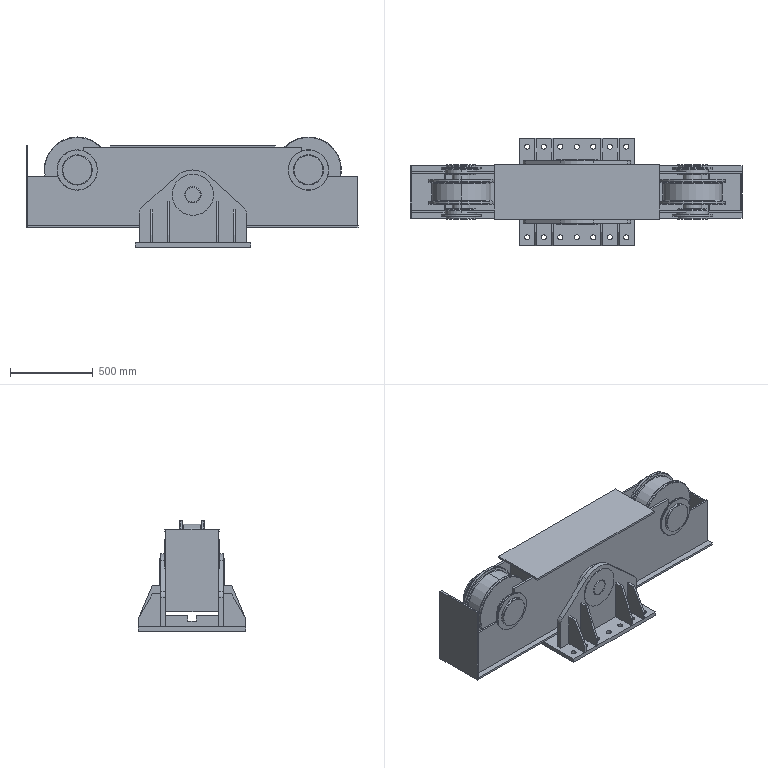Assembly | SolidWorks | mm | 35 component files | 35 solids | 454 faces | box 2010 x 650 x 667 mm | volume 110536923 mm3 | plane 220 | cylinder 134 | torus 72 | cone 28 | commonest cylinder face diameters 100 x30 31 x28 250 x16 195 x14 180 x8 245 x8 240 x8 112 x8
Bill of materials:
700X650X25 | 1 | Plain Carbon Steel | Thin, nearly square flat plate with a single row of seven evenly spaced round through-holes along each of two opposite edges (14 holes total).
Axis | 1 | Plain Carbon Steel | Solid round cylinder (pin or rod shape) with small chamfers or edge breaks at both flat ends.
BottomCover | 1 | Plain Carbon Steel | Thin, plain rectangular flat plate or sheet with no visible holes or cutouts.
Cover1 | 1 | Plain Carbon Steel | Thin, plain rectangular flat plate, taller than it is wide, with no visible features.
Cover2 | 1 | Plain Carbon Steel | Thin, plain rectangular flat plate, close to square, with no visible features. Its thickness ratio is somewhat larger than unnamed part.
FlangeRib1 | 4 | Plain Carbon Steel | Flat plate with a four-sided outline: three square corners and one side cut at an angle, giving a trapezoid with a short vertical edge at the low end.
FlangeRib2 | 4 | Plain Carbon Steel | Flat trapezoidal plate like unnamed part: a straight top, base and one vertical side, plus a long slanted edge that ends in a short vertical edge. It is narrower and slightly steeper than that part.
RibPlate1 | 2 | Plain Carbon Steel | Rectangular flat bar or strip, long compared with its height, with a moderate thickness and no visible holes.
RibPlate2 | 4 | Plain Carbon Steel | Very thin, plain rectangular sheet or plate, taller than it is wide, with no visible features.
SidePlate | 2 | Plain Carbon Steel | Thin, long flat strip with a narrower raised centre section. At each step between the wide and narrow sections there is a rounded, keyhole-like notch, and there is one small round through-hole in the middle.
Support1 | 2 | Plain Carbon Steel | Flat tab or lug plate: a rectangular base with two angled sides rising to a rounded top, small rounded shoulder corners, and one round through-hole near the top.
Support2 | 2 | Plain Carbon Steel | Thin flat ring (washer-like annulus) with a concentric central through-hole.
Support3 | 4 | Plain Carbon Steel | Thin flat circular ring (plain washer-like annulus) with a concentric through-hole; plain flat faces, square edges.
Support4 | 2 | Plain Carbon Steel | Flat circular ring with a concentric through-hole, like part-9d640c60 but visibly thicker; plain flat faces.
Support5 | 1 | Plain Carbon Steel | Rectangular prismatic bar with one rectangular notch cut across its full width at mid-length on one long face.
TopCover | 1 | Plain Carbon Steel | Thin flat rectangular strip or plate with plain rectangular outline; no holes or cutouts visible.
WheelFrom | 2 | Plain Carbon Steel | Rotationally symmetric spool or flanged-roller shape: a central cylindrical drum between two thin end flanges, with a smaller stepped hub sticking out on each side. Each hub ends in a flanged collar.
Mates:
1. coincident | TopCover-1 face at (1250.579, 1256.349, 1665.088) dir (0, 0, 1) | SidePlate-1 face at (2250.579, 1381.349, 1665.088) dir (0, 0, -1)
2. distance | SidePlate-1 face at (1950.579, 1381.349, 2003.088) dir (0, 1, 0) | TopCover-1 face at (250.579, 1416.349, 1653.088) dir (0, 1, 0)
3. coincident | TopCover-1 face at (250.579, 1416.349, 1653.088) dir (-1, 0, 0) | SidePlate-1 face at (250.579, 1381.349, 1665.088) dir (-1, 0, 0)
4. coincident | TopCover-1 face at (250.579, 1416.349, 1653.088) dir (-1, 0, 0) | Cover1-1 face at (250.579, 1256.349, 1903.088) dir (1, 0, 0)
5. coincident | TopCover-1 face at (1250.579, 1256.349, 1653.088) dir (0, 0, -1) | Cover1-1 face at (240.579, 1096.349, 1653.088) dir (0, 0, -1)
6. coincident | TopCover-1 face at (250.579, 1096.349, 1653.088) dir (0, -1, 0) | Cover1-1 face at (240.579, 1096.349, 2153.088) dir (0, -1, 0)
7. coincident | TopCover-1 face at (2250.579, 1416.349, 1653.088) dir (1, 0, 0) | Cover2-1 face at (2250.579, 1256.349, 1809.088) dir (1, 0, 0)
8. coincident | TopCover-1 face at (1250.579, 1256.349, 1665.088) dir (0, 0, 1) | Cover2-1 face at (2250.579, 1143.349, 1665.088) dir (0, 0, -1)
9. coincident | SidePlate-2 face at (1950.579, 1143.349, 2003.088) dir (0, 1, 0) | Cover2-1 face at (2250.579, 1143.349, 1665.088) dir (0, -1, 0)
10. coincident | TopCover-1 face at (1250.579, 1256.349, 1665.088) dir (0, 0, 1) | RibPlate1-1 face at (446.579, 1143.349, 1665.088) dir (0, 0, -1)
11. coincident | SidePlate-1 face at (1950.579, 1369.349, 2003.088) dir (0, -1, 0) | RibPlate1-1 face at (446.579, 1369.349, 1745.088) dir (0, 1, 0)
12. distance | RibPlate1-1 face at (446.579, 1248.002, 1584.123) dir (-1, 0, 0) | Cover1-1 face at (250.579, 1256.349, 1903.088) dir (1, 0, 0)
13. coincident | TopCover-1 face at (1250.579, 1256.349, 1665.088) dir (0, 0, 1) | RibPlate2-1 face at (800.579, 1143.349, 1665.088) dir (0, 0, -1)
14. coincident | SidePlate-1 face at (1950.579, 1369.349, 2003.088) dir (0, -1, 0) | RibPlate2-1 face at (800.579, 1369.349, 1665.088) dir (0, 1, 0)
15. distance | RibPlate2-1 face at (800.579, 1256.349, 1903.088) dir (-1, 0, 0) | Cover1-1 face at (250.579, 1256.349, 1903.088) dir (1, 0, 0)
16. distance | RibPlate2-2 face at (1100.579, 1256.349, 1903.088) dir (-1, 0, 0) | RibPlate2-1 face at (806.579, 1256.349, 1903.088) dir (1, 0, 0)
17. coincident | TopCover-1 face at (1250.579, 1256.349, 1665.088) dir (0, 0, 1) | RibPlate2-2 face at (1100.579, 1143.349, 1665.088) dir (0, 0, -1)
18. coincident | SidePlate-1 face at (1950.579, 1369.349, 2003.088) dir (0, -1, 0) | RibPlate2-2 face at (1100.579, 1369.349, 1665.088) dir (0, 1, 0)
19. coincident | SidePlate-1 face at (1910.579, 1381.349, 2141.088) dir (0, 0, 1) | BottomCover-1 face at (1250.579, 1256.349, 2141.088) dir (0, 0, -1)
20. distance | BottomCover-1 face at (750.579, 1421.349, 2141.088) dir (0, 1, 0) | SidePlate-1 face at (1950.579, 1381.349, 2003.088) dir (0, 1, 0)
21. coincident | BottomCover-1 edge at (1250.579, 1421.349, 2141.088) dir (1, 0, 0) | assembly plane at (1250.579, 0, 0) dir (1, 0, 0)
22. coincident | SidePlate-1 face at (1950.579, 1381.349, 2003.088) dir (0, 1, 0) | Support4-1 face at (1250.579, 1381.349, 1853.088) dir (0, -1, 0)
23. concentric | SidePlate-1 face at (1250.579, 1381.349, 1853.088) dir (0, -1, 0) r 50 | Support4-1 face at (1250.579, 1399.349, 1853.088) dir (0, -1, 0) r 50
24. coincident | SidePlate-2 face at (1950.579, 1131.349, 2003.088) dir (0, -1, 0) | Support4-2 face at (1250.579, 1131.349, 1853.088) dir (0, 1, 0)
25. concentric | SidePlate-2 face at (1250.579, 1143.349, 1853.088) dir (0, -1, 0) r 50 | Support4-2 face at (1250.579, 1131.349, 1853.088) dir (0, -1, 0) r 50
26. coincident | SidePlate-2 face at (1950.579, 1143.349, 2003.088) dir (0, 1, 0) | Support3-1 face at (1250.579, 1143.349, 1853.088) dir (0, -1, 0)
27. concentric | SidePlate-2 face at (1250.579, 1143.349, 1853.088) dir (0, -1, 0) r 50 | Support3-1 face at (1250.579, 1143.349, 1853.088) dir (0, 1, 0) r 50
28. coincident | SidePlate-1 face at (1950.579, 1369.349, 2003.088) dir (0, -1, 0) | Support3-2 face at (1250.579, 1369.349, 1853.088) dir (0, 1, 0)
29. concentric | SidePlate-1 face at (1250.579, 1381.349, 1853.088) dir (0, -1, 0) r 50 | Support3-2 face at (1250.579, 1359.349, 1853.088) dir (0, 1, 0) r 50
30. coincident | TopCover-1 face at (250.579, 1096.349, 1653.088) dir (0, -1, 0) | Support1-1 face at (975.579, 1096.349, 1738.916) dir (0, 1, 0)
31. concentric | SidePlate-2 face at (1250.579, 1143.349, 1853.088) dir (0, -1, 0) r 50 | Support1-1 face at (1250.579, 1066.349, 1853.088) dir (0, 1, 0) r 50
32. parallel | TopCover-1 face at (1250.579, 1256.349, 1653.088) dir (0, 0, -1) | Support1-1 face at (925.579, 1066.349, 1561.088) dir (0, 0, -1)
33. coincident | Support1-1 face at (975.579, 1096.349, 1738.916) dir (0, 1, 0) | Support3-3 face at (1250.579, 1096.349, 1853.088) dir (0, -1, 0)
34. concentric | Support1-1 face at (1250.579, 1066.349, 1853.088) dir (0, 1, 0) r 50 | Support3-3 face at (1250.579, 1096.349, 1853.088) dir (0, 1, 0) r 50
35. coincident | Support1-1 face at (975.579, 1066.349, 1738.916) dir (0, -1, 0) | Support2-1 face at (1250.579, 1066.349, 1853.088) dir (0, 1, 0)
36. concentric | Support1-1 face at (1250.579, 1066.349, 1853.088) dir (0, 1, 0) r 50 | Support2-1 face at (1250.579, 1061.349, 1853.088) dir (0, 1, 0) r 50
37. coincident | Support1-2 face at (925.579, 1416.349, 1561.088) dir (0, 0, -1) | 700X650X25-1 face at (1250.579, 1256.349, 1561.088) dir (0, 0, 1)
38. distance | Support1-1 face at (975.579, 1066.349, 1738.916) dir (0, -1, 0) | 700X650X25-1 face at (900.579, 931.349, 1536.088) dir (0, -1, 0)
39. distance | Support1-1 face at (925.579, 1066.349, 1561.088) dir (-1, 0, 0) | 700X650X25-1 face at (900.579, 1581.349, 1536.088) dir (-1, 0, 0)
40. coincident | 700X650X25-1 face at (1250.579, 1256.349, 1561.088) dir (0, 0, 1) | Support5-1 face at (1235.579, 1416.349, 1561.088) dir (0, 0, -1)
41. coincident | Support1-2 face at (975.579, 1416.349, 1738.916) dir (0, -1, 0) | Support5-1 face at (1235.579, 1416.349, 1561.088) dir (0, 1, 0)
42. coincident | Support5-1 edge at (1250.579, 1096.349, 1561.088) dir (1, 0, 0) | assembly plane at (1250.579, 0, 0) dir (1, 0, 0)
43. coincident | Support1-1 face at (975.579, 1066.349, 1738.916) dir (0, -1, 0) | FlangeRib1-1 face at (1506.579, 1066.349, 1561.088) dir (0, 1, 0)
44. coincident | 700X650X25-1 face at (1250.579, 1256.349, 1561.088) dir (0, 0, 1) | FlangeRib1-1 face at (1506.579, 931.349, 1561.088) dir (0, 0, -1)
45. distance | FlangeRib1-1 face at (1506.579, 931.349, 1561.088) dir (1, 0, 0) | Support1-1 face at (1575.579, 1066.349, 1561.088) dir (1, 0, 0)
46. coincident | Support1-1 face at (975.579, 1066.349, 1738.916) dir (0, -1, 0) | FlangeRib2-1 face at (1406.579, 1066.349, 1561.088) dir (0, 1, 0)
47. coincident | 700X650X25-1 face at (1250.579, 1256.349, 1561.088) dir (0, 0, 1) | FlangeRib2-1 face at (1406.579, 931.349, 1561.088) dir (0, 0, -1)
48. distance | FlangeRib2-1 face at (1406.579, 931.349, 1561.088) dir (1, 0, 0) | FlangeRib1-1 face at (1494.579, 931.349, 1561.088) dir (-1, 0, 0)
49. concentric | SidePlate-2 face at (550.579, 1143.349, 2003.088) dir (0, -1, 0) r 97.5 | WheelFrom-3 face at (550.579, 1647.349, 2003.088) dir (0, 1, 0) r 97.5
50. distance | SidePlate-2 face at (1950.579, 1131.349, 2003.088) dir (0, -1, 0) | WheelFrom-3 face at (550.579, 1121.349, 2123.088) dir (0, 1, 0)
51. concentric | SidePlate-1 face at (1950.579, 1381.349, 2003.088) dir (0, -1, 0) r 97.5 | WheelFrom-4 face at (1950.579, 1647.349, 2003.088) dir (0, 1, 0) r 97.5
52. distance | WheelFrom-4 face at (1830.579, 1391.349, 2003.088) dir (0, -1, 0) | SidePlate-1 face at (1950.579, 1381.349, 2003.088) dir (0, 1, 0)
53. concentric | Support1-1 face at (1250.579, 1066.349, 1853.088) dir (0, 1, 0) r 50 | Axis-1 face at (1250.579, 1451.349, 1853.088) dir (0, -1, 0) r 50
54. coincident | Support2-1 face at (1250.579, 1061.349, 1853.088) dir (0, -1, 0) | Axis-1 face at (1250.579, 1061.349, 1853.088) dir (0, -1, 0)